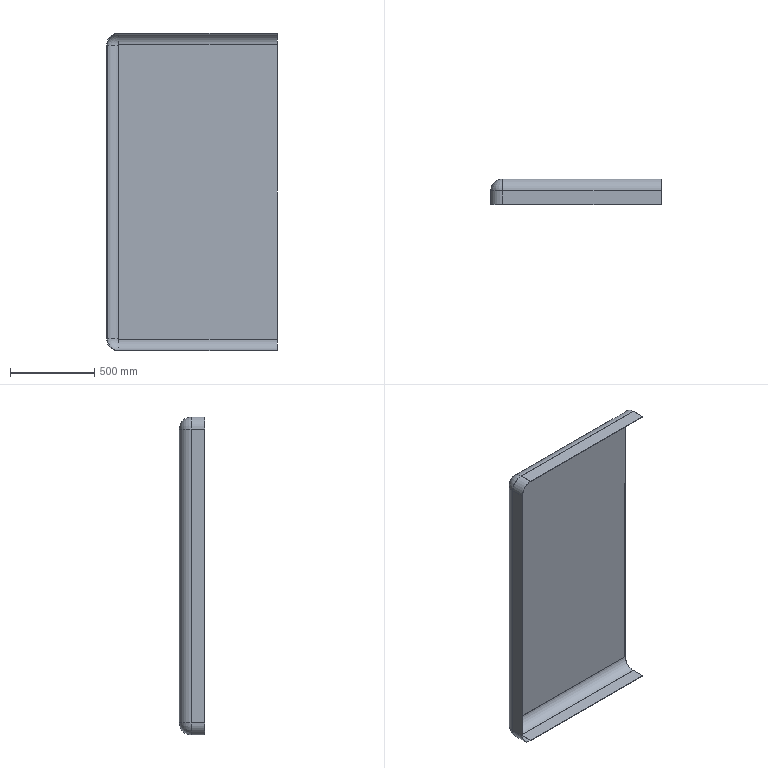Component | SolidWorks | TopHousingAssembly-1_CasingA-1 | 1 solid | 28 faces | box 1009.5 x 149.5 x 1881 mm | volume 7036738 mm3 | plane 14 | cylinder 10 | torus 4 | commonest cylinder face diameters 139 x3 133 x3 141 x2 135 x2
STEP:
#1=CARTESIAN_POINT('',(-0.2362,96.791,71.201));
#2=VERTEX_POINT('',#1);
#3=CARTESIAN_POINT('',(-0.2362,96.909,71.201));
#4=VERTEX_POINT('',#3);
#5=CARTESIAN_POINT('',(-0.2362,96.909,71.201));
#6=DIRECTION('',(0.,1.,0.));
#7=VECTOR('',#6,39.37);
#8=LINE('',#5,#7);
#9=EDGE_CURVE('',#2,#4,#8,.T.);
#10=ORIENTED_EDGE('',*,*,#9,.F.);
#11=CARTESIAN_POINT('',(-0.2362,96.791,2.618));
#12=VERTEX_POINT('',#11);
#13=CARTESIAN_POINT('',(-0.2362,96.791,36.909));
#14=DIRECTION('',(0.,0.,-1.));
#15=VECTOR('',#14,39.37);
#16=LINE('',#13,#15);
#17=EDGE_CURVE('',#2,#12,#16,.T.);
#18=ORIENTED_EDGE('',*,*,#17,.T.);
#19=CARTESIAN_POINT('',(-0.2362,96.909,2.618));
#20=VERTEX_POINT('',#19);
#21=CARTESIAN_POINT('',(-0.2362,96.909,2.618));
#22=DIRECTION('',(0.,1.,0.));
#23=VECTOR('',#22,39.37);
#24=LINE('',#21,#23);
#25=EDGE_CURVE('',#12,#20,#24,.T.);
#26=ORIENTED_EDGE('',*,*,#25,.T.);
#27=CARTESIAN_POINT('',(-0.2362,96.909,71.201));
#28=DIRECTION('',(0.,0.,-1.));
#29=VECTOR('',#28,39.37);
#30=LINE('',#27,#29);
#31=EDGE_CURVE('',#4,#20,#30,.T.);
#32=ORIENTED_EDGE('',*,*,#31,.F.);
#33=EDGE_LOOP('',(#10,#18,#26,#32));
#34=FACE_OUTER_BOUND('',#33,.T.);
#35=CARTESIAN_POINT('',(-0.2362,96.909,71.201));
#36=DIRECTION('',(-1.,0.,0.));
#37=DIRECTION('',(0.,0.,-1.));
#38=AXIS2_PLACEMENT_3D('',#35,#36,#37);
#39=PLANE('',#38);
#40=ADVANCED_FACE('',(#34),#39,.F.);
#41=CARTESIAN_POINT('',(-37.244,96.909,2.657));
#42=VERTEX_POINT('',#41);
#43=CARTESIAN_POINT('',(-37.244,96.909,71.161));
#44=VERTEX_POINT('',#43);
#45=CARTESIAN_POINT('',(-37.244,96.909,71.201));
#46=DIRECTION('',(0.,0.,1.));
#47=VECTOR('',#46,39.37);
#48=LINE('',#45,#47);
#49=EDGE_CURVE('',#42,#44,#48,.T.);
#50=ORIENTED_EDGE('',*,*,#49,.T.);
#51=CARTESIAN_POINT('',(-37.205,96.909,71.201));
#52=VERTEX_POINT('',#51);
#53=CARTESIAN_POINT('',(-37.205,96.909,71.161));
#54=DIRECTION('',(0.,1.,0.));
#55=DIRECTION('',(0.,0.,-1.));
#56=AXIS2_PLACEMENT_3D('',#53,#54,#55);
#57=CIRCLE('',#56,0.03937);
#58=EDGE_CURVE('',#44,#52,#57,.T.);
#59=ORIENTED_EDGE('',*,*,#58,.T.);
#60=CARTESIAN_POINT('',(-37.244,96.909,71.201));
#61=DIRECTION('',(1.,0.,0.));
#62=VECTOR('',#61,39.37);
#63=LINE('',#60,#62);
#64=EDGE_CURVE('',#52,#4,#63,.T.);
#65=ORIENTED_EDGE('',*,*,#64,.T.);
#66=ORIENTED_EDGE('',*,*,#31,.T.);
#67=CARTESIAN_POINT('',(-37.205,96.909,2.618));
#68=VERTEX_POINT('',#67);
#69=CARTESIAN_POINT('',(-37.244,96.909,2.618));
#70=DIRECTION('',(-1.,0.,0.));
#71=VECTOR('',#70,39.37);
#72=LINE('',#69,#71);
#73=EDGE_CURVE('',#20,#68,#72,.T.);
#74=ORIENTED_EDGE('',*,*,#73,.T.);
#75=CARTESIAN_POINT('',(-37.205,96.909,2.657));
#76=DIRECTION('',(0.,1.,0.));
#77=DIRECTION('',(0.,0.,-1.));
#78=AXIS2_PLACEMENT_3D('',#75,#76,#77);
#79=CIRCLE('',#78,0.03937);
#80=EDGE_CURVE('',#68,#42,#79,.T.);
#81=ORIENTED_EDGE('',*,*,#80,.T.);
#82=EDGE_LOOP('',(#50,#59,#65,#66,#74,#81));
#83=FACE_OUTER_BOUND('',#82,.T.);
#84=CARTESIAN_POINT('',(-18.74,96.909,36.909));
#85=DIRECTION('',(0.,-1.,0.));
#86=DIRECTION('',(0.,0.,-1.));
#87=AXIS2_PLACEMENT_3D('',#84,#85,#86);
#88=PLANE('',#87);
#89=ADVANCED_FACE('',(#83),#88,.F.);
#90=CARTESIAN_POINT('',(-37.205,96.791,71.201));
#91=VERTEX_POINT('',#90);
#92=CARTESIAN_POINT('',(-18.74,96.791,71.201));
#93=DIRECTION('',(1.,0.,0.));
#94=VECTOR('',#93,39.37);
#95=LINE('',#92,#94);
#96=EDGE_CURVE('',#91,#2,#95,.T.);
#97=ORIENTED_EDGE('',*,*,#96,.F.);
#98=CARTESIAN_POINT('',(-37.244,96.791,71.161));
#99=VERTEX_POINT('',#98);
#100=CARTESIAN_POINT('',(-37.205,96.791,71.161));
#101=DIRECTION('',(0.,-1.,0.));
#102=DIRECTION('',(0.,0.,-1.));
#103=AXIS2_PLACEMENT_3D('',#100,#101,#102);
#104=CIRCLE('',#103,0.03937);
#105=EDGE_CURVE('',#91,#99,#104,.T.);
#106=ORIENTED_EDGE('',*,*,#105,.T.);
#107=CARTESIAN_POINT('',(-37.244,96.791,2.657));
#108=VERTEX_POINT('',#107);
#109=CARTESIAN_POINT('',(-37.244,96.791,36.909));
#110=DIRECTION('',(0.,0.,1.));
#111=VECTOR('',#110,39.37);
#112=LINE('',#109,#111);
#113=EDGE_CURVE('',#108,#99,#112,.T.);
#114=ORIENTED_EDGE('',*,*,#113,.F.);
#115=CARTESIAN_POINT('',(-37.205,96.791,2.618));
#116=VERTEX_POINT('',#115);
#117=CARTESIAN_POINT('',(-37.205,96.791,2.657));
#118=DIRECTION('',(0.,-1.,0.));
#119=DIRECTION('',(0.,0.,-1.));
#120=AXIS2_PLACEMENT_3D('',#117,#118,#119);
#121=CIRCLE('',#120,0.03937);
#122=EDGE_CURVE('',#108,#116,#121,.T.);
#123=ORIENTED_EDGE('',*,*,#122,.T.);
#124=CARTESIAN_POINT('',(-18.74,96.791,2.618));
#125=DIRECTION('',(-1.,0.,0.));
#126=VECTOR('',#125,39.37);
#127=LINE('',#124,#126);
#128=EDGE_CURVE('',#12,#116,#127,.T.);
#129=ORIENTED_EDGE('',*,*,#128,.F.);
#130=ORIENTED_EDGE('',*,*,#17,.F.);
#131=EDGE_LOOP('',(#97,#106,#114,#123,#129,#130));
#132=FACE_OUTER_BOUND('',#131,.T.);
#133=CARTESIAN_POINT('',(-18.74,96.791,36.909));
#134=DIRECTION('',(0.,-1.,0.));
#135=DIRECTION('',(0.,0.,-1.));
#136=AXIS2_PLACEMENT_3D('',#133,#134,#135);
#137=PLANE('',#136);
#138=ADVANCED_FACE('',(#132),#137,.T.);
#139=CARTESIAN_POINT('',(-0.2362,94.173,73.819));
#140=VERTEX_POINT('',#139);
#141=CARTESIAN_POINT('',(-0.2362,94.173,73.937));
#142=VERTEX_POINT('',#141);
#143=CARTESIAN_POINT('',(-0.2362,94.173,73.937));
#144=DIRECTION('',(0.,0.,1.));
#145=VECTOR('',#144,39.37);
#146=LINE('',#143,#145);
#147=EDGE_CURVE('',#140,#142,#146,.T.);
#148=ORIENTED_EDGE('',*,*,#147,.F.);
#149=CARTESIAN_POINT('',(-0.2362,94.173,71.201));
#150=DIRECTION('',(1.,0.,0.));
#151=DIRECTION('',(0.,-0.,1.));
#152=AXIS2_PLACEMENT_3D('',#149,#150,#151);
#153=CIRCLE('',#152,2.618);
#154=EDGE_CURVE('',#2,#140,#153,.T.);
#155=ORIENTED_EDGE('',*,*,#154,.F.);
#156=ORIENTED_EDGE('',*,*,#9,.T.);
#157=CARTESIAN_POINT('',(-0.2362,94.173,71.201));
#158=DIRECTION('',(1.,0.,0.));
#159=DIRECTION('',(0.,-0.,1.));
#160=AXIS2_PLACEMENT_3D('',#157,#158,#159);
#161=CIRCLE('',#160,2.736);
#162=EDGE_CURVE('',#4,#142,#161,.T.);
#163=ORIENTED_EDGE('',*,*,#162,.T.);
#164=EDGE_LOOP('',(#148,#155,#156,#163));
#165=FACE_OUTER_BOUND('',#164,.T.);
#166=CARTESIAN_POINT('',(-0.2362,94.173,71.201));
#167=DIRECTION('',(1.,0.,0.));
#168=DIRECTION('',(0.,0.,-1.));
#169=AXIS2_PLACEMENT_3D('',#166,#167,#168);
#170=PLANE('',#169);
#171=ADVANCED_FACE('',(#165),#170,.T.);
#172=ORIENTED_EDGE('',*,*,#64,.F.);
#173=CARTESIAN_POINT('',(-37.205,94.173,73.937));
#174=VERTEX_POINT('',#173);
#175=CARTESIAN_POINT('',(-37.205,94.173,71.201));
#176=DIRECTION('',(-1.,0.,0.));
#177=DIRECTION('',(0.,0.,1.));
#178=AXIS2_PLACEMENT_3D('',#175,#176,#177);
#179=CIRCLE('',#178,2.736);
#180=EDGE_CURVE('',#174,#52,#179,.T.);
#181=ORIENTED_EDGE('',*,*,#180,.F.);
#182=CARTESIAN_POINT('',(-0.2362,94.173,73.937));
#183=DIRECTION('',(1.,0.,0.));
#184=VECTOR('',#183,39.37);
#185=LINE('',#182,#184);
#186=EDGE_CURVE('',#174,#142,#185,.T.);
#187=ORIENTED_EDGE('',*,*,#186,.T.);
#188=ORIENTED_EDGE('',*,*,#162,.F.);
#189=EDGE_LOOP('',(#172,#181,#187,#188));
#190=FACE_OUTER_BOUND('',#189,.T.);
#191=CARTESIAN_POINT('',(-37.205,94.173,71.201));
#192=DIRECTION('',(-1.,0.,0.));
#193=DIRECTION('',(0.,0.,1.));
#194=AXIS2_PLACEMENT_3D('',#191,#192,#193);
#195=CYLINDRICAL_SURFACE('',#194,2.736);
#196=ADVANCED_FACE('',(#190),#195,.T.);
#197=ORIENTED_EDGE('',*,*,#96,.T.);
#198=ORIENTED_EDGE('',*,*,#154,.T.);
#199=CARTESIAN_POINT('',(-37.205,94.173,73.819));
#200=VERTEX_POINT('',#199);
#201=CARTESIAN_POINT('',(-0.2362,94.173,73.819));
#202=DIRECTION('',(-1.,0.,0.));
#203=VECTOR('',#202,39.37);
#204=LINE('',#201,#203);
#205=EDGE_CURVE('',#140,#200,#204,.T.);
#206=ORIENTED_EDGE('',*,*,#205,.T.);
#207=CARTESIAN_POINT('',(-37.205,94.173,71.201));
#208=DIRECTION('',(-1.,0.,0.));
#209=DIRECTION('',(0.,0.,1.));
#210=AXIS2_PLACEMENT_3D('',#207,#208,#209);
#211=CIRCLE('',#210,2.618);
#212=EDGE_CURVE('',#200,#91,#211,.T.);
#213=ORIENTED_EDGE('',*,*,#212,.T.);
#214=EDGE_LOOP('',(#197,#198,#206,#213));
#215=FACE_OUTER_BOUND('',#214,.T.);
#216=CARTESIAN_POINT('',(-37.205,94.173,71.201));
#217=DIRECTION('',(-1.,0.,0.));
#218=DIRECTION('',(0.,0.,1.));
#219=AXIS2_PLACEMENT_3D('',#216,#217,#218);
#220=CYLINDRICAL_SURFACE('',#219,2.618);
#221=ADVANCED_FACE('',(#215),#220,.F.);
#222=ORIENTED_EDGE('',*,*,#147,.T.);
#223=CARTESIAN_POINT('',(-0.2362,91.024,73.937));
#224=VERTEX_POINT('',#223);
#225=CARTESIAN_POINT('',(-0.2362,96.791,73.937));
#226=DIRECTION('',(-0.,1.,-0.));
#227=VECTOR('',#226,39.37);
#228=LINE('',#225,#227);
#229=EDGE_CURVE('',#224,#142,#228,.T.);
#230=ORIENTED_EDGE('',*,*,#229,.F.);
#231=CARTESIAN_POINT('',(-0.2362,91.024,73.819));
#232=VERTEX_POINT('',#231);
#233=CARTESIAN_POINT('',(-0.2362,91.024,73.937));
#234=DIRECTION('',(0.,-0.,-1.));
#235=VECTOR('',#234,39.37);
#236=LINE('',#233,#235);
#237=EDGE_CURVE('',#224,#232,#236,.T.);
#238=ORIENTED_EDGE('',*,*,#237,.T.);
#239=CARTESIAN_POINT('',(-0.2362,96.791,73.819));
#240=DIRECTION('',(-0.,1.,-0.));
#241=VECTOR('',#240,39.37);
#242=LINE('',#239,#241);
#243=EDGE_CURVE('',#232,#140,#242,.T.);
#244=ORIENTED_EDGE('',*,*,#243,.T.);
#245=EDGE_LOOP('',(#222,#230,#238,#244));
#246=FACE_OUTER_BOUND('',#245,.T.);
#247=CARTESIAN_POINT('',(-0.2362,96.791,73.937));
#248=DIRECTION('',(-1.,-0.,0.));
#249=DIRECTION('',(0.,-1.,0.));
#250=AXIS2_PLACEMENT_3D('',#247,#248,#249);
#251=PLANE('',#250);
#252=ADVANCED_FACE('',(#246),#251,.F.);
#253=ORIENTED_EDGE('',*,*,#186,.F.);
#254=CARTESIAN_POINT('',(-37.205,91.024,73.937));
#255=VERTEX_POINT('',#254);
#256=CARTESIAN_POINT('',(-37.205,96.791,73.937));
#257=DIRECTION('',(0.,-1.,0.));
#258=VECTOR('',#257,39.37);
#259=LINE('',#256,#258);
#260=EDGE_CURVE('',#174,#255,#259,.T.);
#261=ORIENTED_EDGE('',*,*,#260,.T.);
#262=CARTESIAN_POINT('',(-18.74,91.024,73.937));
#263=DIRECTION('',(1.,0.,0.));
#264=VECTOR('',#263,39.37);
#265=LINE('',#262,#264);
#266=EDGE_CURVE('',#255,#224,#265,.T.);
#267=ORIENTED_EDGE('',*,*,#266,.T.);
#268=ORIENTED_EDGE('',*,*,#229,.T.);
#269=EDGE_LOOP('',(#253,#261,#267,#268));
#270=FACE_OUTER_BOUND('',#269,.T.);
#271=CARTESIAN_POINT('',(-18.74,96.791,73.937));
#272=DIRECTION('',(0.,-0.,-1.));
#273=DIRECTION('',(0.,1.,-0.));
#274=AXIS2_PLACEMENT_3D('',#271,#272,#273);
#275=PLANE('',#274);
#276=ADVANCED_FACE('',(#270),#275,.F.);
#277=CARTESIAN_POINT('',(-37.205,91.024,73.819));
#278=VERTEX_POINT('',#277);
#279=CARTESIAN_POINT('',(-37.205,91.024,73.819));
#280=DIRECTION('',(0.,-1.,0.));
#281=VECTOR('',#280,39.37);
#282=LINE('',#279,#281);
#283=EDGE_CURVE('',#200,#278,#282,.T.);
#284=ORIENTED_EDGE('',*,*,#283,.F.);
#285=ORIENTED_EDGE('',*,*,#205,.F.);
#286=ORIENTED_EDGE('',*,*,#243,.F.);
#287=CARTESIAN_POINT('',(-0.2362,91.024,73.819));
#288=DIRECTION('',(1.,0.,0.));
#289=VECTOR('',#288,39.37);
#290=LINE('',#287,#289);
#291=EDGE_CURVE('',#278,#232,#290,.T.);
#292=ORIENTED_EDGE('',*,*,#291,.F.);
#293=EDGE_LOOP('',(#284,#285,#286,#292));
#294=FACE_OUTER_BOUND('',#293,.T.);
#295=CARTESIAN_POINT('',(-18.74,96.791,73.819));
#296=DIRECTION('',(0.,-0.,-1.));
#297=DIRECTION('',(0.,1.,-0.));
#298=AXIS2_PLACEMENT_3D('',#295,#296,#297);
#299=PLANE('',#298);
#300=ADVANCED_FACE('',(#294),#299,.T.);
#301=ORIENTED_EDGE('',*,*,#291,.T.);
#302=ORIENTED_EDGE('',*,*,#237,.F.);
#303=ORIENTED_EDGE('',*,*,#266,.F.);
#304=CARTESIAN_POINT('',(-39.98,91.024,71.161));
#305=VERTEX_POINT('',#304);
#306=CARTESIAN_POINT('',(-37.205,91.024,71.161));
#307=DIRECTION('',(0.,-1.,0.));
#308=DIRECTION('',(0.,0.,1.));
#309=AXIS2_PLACEMENT_3D('',#306,#307,#308);
#310=CIRCLE('',#309,2.776);
#311=EDGE_CURVE('',#255,#305,#310,.T.);
#312=ORIENTED_EDGE('',*,*,#311,.T.);
#313=CARTESIAN_POINT('',(-39.98,91.024,2.657));
#314=VERTEX_POINT('',#313);
#315=CARTESIAN_POINT('',(-39.98,91.024,36.909));
#316=DIRECTION('',(0.,0.,1.));
#317=VECTOR('',#316,39.37);
#318=LINE('',#315,#317);
#319=EDGE_CURVE('',#314,#305,#318,.T.);
#320=ORIENTED_EDGE('',*,*,#319,.F.);
#321=CARTESIAN_POINT('',(-37.205,91.024,-0.1181));
#322=VERTEX_POINT('',#321);
#323=CARTESIAN_POINT('',(-37.205,91.024,2.657));
#324=DIRECTION('',(0.,-1.,0.));
#325=DIRECTION('',(-1.,0.,0.));
#326=AXIS2_PLACEMENT_3D('',#323,#324,#325);
#327=CIRCLE('',#326,2.776);
#328=EDGE_CURVE('',#314,#322,#327,.T.);
#329=ORIENTED_EDGE('',*,*,#328,.T.);
#330=CARTESIAN_POINT('',(-0.2362,91.024,-0.1181));
#331=VERTEX_POINT('',#330);
#332=CARTESIAN_POINT('',(-18.74,91.024,-0.1181));
#333=DIRECTION('',(-1.,0.,0.));
#334=VECTOR('',#333,39.37);
#335=LINE('',#332,#334);
#336=EDGE_CURVE('',#331,#322,#335,.T.);
#337=ORIENTED_EDGE('',*,*,#336,.F.);
#338=CARTESIAN_POINT('',(-0.2362,91.024,-0.));
#339=VERTEX_POINT('',#338);
#340=CARTESIAN_POINT('',(-0.2362,91.024,-0.1181));
#341=DIRECTION('',(0.,-0.,1.));
#342=VECTOR('',#341,39.37);
#343=LINE('',#340,#342);
#344=EDGE_CURVE('',#331,#339,#343,.T.);
#345=ORIENTED_EDGE('',*,*,#344,.T.);
#346=CARTESIAN_POINT('',(-37.205,91.024,-0.));
#347=VERTEX_POINT('',#346);
#348=CARTESIAN_POINT('',(-37.205,91.024,-0.));
#349=DIRECTION('',(-1.,0.,0.));
#350=VECTOR('',#349,39.37);
#351=LINE('',#348,#350);
#352=EDGE_CURVE('',#339,#347,#351,.T.);
#353=ORIENTED_EDGE('',*,*,#352,.T.);
#354=CARTESIAN_POINT('',(-39.862,91.024,2.657));
#355=VERTEX_POINT('',#354);
#356=CARTESIAN_POINT('',(-37.205,91.024,2.657));
#357=DIRECTION('',(0.,-1.,0.));
#358=DIRECTION('',(-1.,0.,0.));
#359=AXIS2_PLACEMENT_3D('',#356,#357,#358);
#360=CIRCLE('',#359,2.657);
#361=EDGE_CURVE('',#355,#347,#360,.T.);
#362=ORIENTED_EDGE('',*,*,#361,.F.);
#363=CARTESIAN_POINT('',(-39.862,91.024,71.161));
#364=VERTEX_POINT('',#363);
#365=CARTESIAN_POINT('',(-39.862,91.024,71.161));
#366=DIRECTION('',(0.,0.,1.));
#367=VECTOR('',#366,39.37);
#368=LINE('',#365,#367);
#369=EDGE_CURVE('',#355,#364,#368,.T.);
#370=ORIENTED_EDGE('',*,*,#369,.T.);
#371=CARTESIAN_POINT('',(-37.205,91.024,71.161));
#372=DIRECTION('',(0.,-1.,0.));
#373=DIRECTION('',(0.,0.,1.));
#374=AXIS2_PLACEMENT_3D('',#371,#372,#373);
#375=CIRCLE('',#374,2.657);
#376=EDGE_CURVE('',#278,#364,#375,.T.);
#377=ORIENTED_EDGE('',*,*,#376,.F.);
#378=EDGE_LOOP('',(#301,#302,#303,#312,#320,#329,#337,#345,#353,#362,#370,#377));
#379=FACE_OUTER_BOUND('',#378,.T.);
#380=CARTESIAN_POINT('',(-0.2362,91.024,73.937));
#381=DIRECTION('',(0.,1.,-0.));
#382=DIRECTION('',(0.,0.,1.));
#383=AXIS2_PLACEMENT_3D('',#380,#381,#382);
#384=PLANE('',#383);
#385=ADVANCED_FACE('',(#379),#384,.F.);
#386=ORIENTED_EDGE('',*,*,#49,.F.);
#387=CARTESIAN_POINT('',(-39.98,94.173,2.657));
#388=VERTEX_POINT('',#387);
#389=CARTESIAN_POINT('',(-37.244,94.173,2.657));
#390=DIRECTION('',(0.,0.,-1.));
#391=DIRECTION('',(-1.,0.,0.));
#392=AXIS2_PLACEMENT_3D('',#389,#390,#391);
#393=CIRCLE('',#392,2.736);
#394=EDGE_CURVE('',#388,#42,#393,.T.);
#395=ORIENTED_EDGE('',*,*,#394,.F.);
#396=CARTESIAN_POINT('',(-39.98,94.173,71.161));
#397=VERTEX_POINT('',#396);
#398=CARTESIAN_POINT('',(-39.98,94.173,71.161));
#399=DIRECTION('',(0.,0.,1.));
#400=VECTOR('',#399,39.37);
#401=LINE('',#398,#400);
#402=EDGE_CURVE('',#388,#397,#401,.T.);
#403=ORIENTED_EDGE('',*,*,#402,.T.);
#404=CARTESIAN_POINT('',(-37.244,94.173,71.161));
#405=DIRECTION('',(0.,0.,1.));
#406=DIRECTION('',(-1.,-0.,0.));
#407=AXIS2_PLACEMENT_3D('',#404,#405,#406);
#408=CIRCLE('',#407,2.736);
#409=EDGE_CURVE('',#44,#397,#408,.T.);
#410=ORIENTED_EDGE('',*,*,#409,.F.);
#411=EDGE_LOOP('',(#386,#395,#403,#410));
#412=FACE_OUTER_BOUND('',#411,.T.);
#413=CARTESIAN_POINT('',(-37.244,94.173,2.657));
#414=DIRECTION('',(0.,0.,-1.));
#415=DIRECTION('',(-1.,0.,0.));
#416=AXIS2_PLACEMENT_3D('',#413,#414,#415);
#417=CYLINDRICAL_SURFACE('',#416,2.736);
#418=ADVANCED_FACE('',(#412),#417,.T.);
#419=ORIENTED_EDGE('',*,*,#113,.T.);
#420=CARTESIAN_POINT('',(-39.862,94.173,71.161));
#421=VERTEX_POINT('',#420);
#422=CARTESIAN_POINT('',(-37.244,94.173,71.161));
#423=DIRECTION('',(0.,0.,1.));
#424=DIRECTION('',(-1.,0.,0.));
#425=AXIS2_PLACEMENT_3D('',#422,#423,#424);
#426=CIRCLE('',#425,2.618);
#427=EDGE_CURVE('',#99,#421,#426,.T.);
#428=ORIENTED_EDGE('',*,*,#427,.T.);
#429=CARTESIAN_POINT('',(-39.862,94.173,2.657));
#430=VERTEX_POINT('',#429);
#431=CARTESIAN_POINT('',(-39.862,94.173,71.161));
#432=DIRECTION('',(0.,0.,-1.));
#433=VECTOR('',#432,39.37);
#434=LINE('',#431,#433);
#435=EDGE_CURVE('',#421,#430,#434,.T.);
#436=ORIENTED_EDGE('',*,*,#435,.T.);
#437=CARTESIAN_POINT('',(-37.244,94.173,2.657));
#438=DIRECTION('',(0.,0.,-1.));
#439=DIRECTION('',(-1.,0.,0.));
#440=AXIS2_PLACEMENT_3D('',#437,#438,#439);
#441=CIRCLE('',#440,2.618);
#442=EDGE_CURVE('',#430,#108,#441,.T.);
#443=ORIENTED_EDGE('',*,*,#442,.T.);
#444=EDGE_LOOP('',(#419,#428,#436,#443));
#445=FACE_OUTER_BOUND('',#444,.T.);
#446=CARTESIAN_POINT('',(-37.244,94.173,2.657));
#447=DIRECTION('',(0.,0.,-1.));
#448=DIRECTION('',(-1.,0.,0.));
#449=AXIS2_PLACEMENT_3D('',#446,#447,#448);
#450=CYLINDRICAL_SURFACE('',#449,2.618);
#451=ADVANCED_FACE('',(#445),#450,.F.);
#452=ORIENTED_EDGE('',*,*,#402,.F.);
#453=CARTESIAN_POINT('',(-39.98,96.791,2.657));
#454=DIRECTION('',(-0.,-1.,0.));
#455=VECTOR('',#454,39.37);
#456=LINE('',#453,#455);
#457=EDGE_CURVE('',#388,#314,#456,.T.);
#458=ORIENTED_EDGE('',*,*,#457,.T.);
#459=ORIENTED_EDGE('',*,*,#319,.T.);
#460=CARTESIAN_POINT('',(-39.98,96.791,71.161));
#461=DIRECTION('',(0.,1.,0.));
#462=VECTOR('',#461,39.37);
#463=LINE('',#460,#462);
#464=EDGE_CURVE('',#305,#397,#463,.T.);
#465=ORIENTED_EDGE('',*,*,#464,.T.);
#466=EDGE_LOOP('',(#452,#458,#459,#465));
#467=FACE_OUTER_BOUND('',#466,.T.);
#468=CARTESIAN_POINT('',(-39.98,96.791,36.909));
#469=DIRECTION('',(1.,-0.,0.));
#470=DIRECTION('',(0.,1.,0.));
#471=AXIS2_PLACEMENT_3D('',#468,#469,#470);
#472=PLANE('',#471);
#473=ADVANCED_FACE('',(#467),#472,.F.);
#474=CARTESIAN_POINT('',(-39.862,91.024,2.657));
#475=DIRECTION('',(-0.,-1.,0.));
#476=VECTOR('',#475,39.37);
#477=LINE('',#474,#476);
#478=EDGE_CURVE('',#430,#355,#477,.T.);
#479=ORIENTED_EDGE('',*,*,#478,.F.);
#480=ORIENTED_EDGE('',*,*,#435,.F.);
#481=CARTESIAN_POINT('',(-39.862,96.791,71.161));
#482=DIRECTION('',(0.,1.,0.));
#483=VECTOR('',#482,39.37);
#484=LINE('',#481,#483);
#485=EDGE_CURVE('',#364,#421,#484,.T.);
#486=ORIENTED_EDGE('',*,*,#485,.F.);
#487=ORIENTED_EDGE('',*,*,#369,.F.);
#488=EDGE_LOOP('',(#479,#480,#486,#487));
#489=FACE_OUTER_BOUND('',#488,.T.);
#490=CARTESIAN_POINT('',(-39.862,96.791,36.909));
#491=DIRECTION('',(1.,-0.,0.));
#492=DIRECTION('',(0.,1.,0.));
#493=AXIS2_PLACEMENT_3D('',#490,#491,#492);
#494=PLANE('',#493);
#495=ADVANCED_FACE('',(#489),#494,.T.);
#496=CARTESIAN_POINT('',(-0.2362,94.173,-0.));
#497=VERTEX_POINT('',#496);
#498=CARTESIAN_POINT('',(-0.2362,94.173,2.618));
#499=DIRECTION('',(1.,0.,0.));
#500=DIRECTION('',(0.,0.,-1.));
#501=AXIS2_PLACEMENT_3D('',#498,#499,#500);
#502=CIRCLE('',#501,2.618);
#503=EDGE_CURVE('',#497,#12,#502,.T.);
#504=ORIENTED_EDGE('',*,*,#503,.F.);
#505=CARTESIAN_POINT('',(-0.2362,94.173,-0.1181));
#506=VERTEX_POINT('',#505);
#507=CARTESIAN_POINT('',(-0.2362,94.173,-0.));
#508=DIRECTION('',(0.,0.,-1.));
#509=VECTOR('',#508,39.37);
#510=LINE('',#507,#509);
#511=EDGE_CURVE('',#497,#506,#510,.T.);
#512=ORIENTED_EDGE('',*,*,#511,.T.);
#513=CARTESIAN_POINT('',(-0.2362,94.173,2.618));
#514=DIRECTION('',(1.,0.,0.));
#515=DIRECTION('',(0.,0.,-1.));
#516=AXIS2_PLACEMENT_3D('',#513,#514,#515);
#517=CIRCLE('',#516,2.736);
#518=EDGE_CURVE('',#506,#20,#517,.T.);
#519=ORIENTED_EDGE('',*,*,#518,.T.);
#520=ORIENTED_EDGE('',*,*,#25,.F.);
#521=EDGE_LOOP('',(#504,#512,#519,#520));
#522=FACE_OUTER_BOUND('',#521,.T.);
#523=CARTESIAN_POINT('',(-0.2362,94.173,2.618));
#524=DIRECTION('',(-1.,0.,0.));
#525=DIRECTION('',(0.,0.,1.));
#526=AXIS2_PLACEMENT_3D('',#523,#524,#525);
#527=PLANE('',#526);
#528=ADVANCED_FACE('',(#522),#527,.F.);
#529=ORIENTED_EDGE('',*,*,#73,.F.);
#530=ORIENTED_EDGE('',*,*,#518,.F.);
#531=CARTESIAN_POINT('',(-37.205,94.173,-0.1181));
#532=VERTEX_POINT('',#531);
#533=CARTESIAN_POINT('',(-37.205,94.173,-0.1181));
#534=DIRECTION('',(-1.,0.,0.));
#535=VECTOR('',#534,39.37);
#536=LINE('',#533,#535);
#537=EDGE_CURVE('',#506,#532,#536,.T.);
#538=ORIENTED_EDGE('',*,*,#537,.T.);
#539=CARTESIAN_POINT('',(-37.205,94.173,2.618));
#540=DIRECTION('',(-1.,0.,0.));
#541=DIRECTION('',(0.,-0.,-1.));
#542=AXIS2_PLACEMENT_3D('',#539,#540,#541);
#543=CIRCLE('',#542,2.736);
#544=EDGE_CURVE('',#68,#532,#543,.T.);
#545=ORIENTED_EDGE('',*,*,#544,.F.);
#546=EDGE_LOOP('',(#529,#530,#538,#545));
#547=FACE_OUTER_BOUND('',#546,.T.);
#548=CARTESIAN_POINT('',(-0.2362,94.173,2.618));
#549=DIRECTION('',(1.,0.,0.));
#550=DIRECTION('',(0.,0.,-1.));
#551=AXIS2_PLACEMENT_3D('',#548,#549,#550);
#552=CYLINDRICAL_SURFACE('',#551,2.736);
#553=ADVANCED_FACE('',(#547),#552,.T.);
#554=ORIENTED_EDGE('',*,*,#128,.T.);
#555=CARTESIAN_POINT('',(-37.205,94.173,-0.));
#556=VERTEX_POINT('',#555);
#557=CARTESIAN_POINT('',(-37.205,94.173,2.618));
#558=DIRECTION('',(-1.,0.,0.));
#559=DIRECTION('',(0.,-0.,-1.));
#560=AXIS2_PLACEMENT_3D('',#557,#558,#559);
#561=CIRCLE('',#560,2.618);
#562=EDGE_CURVE('',#116,#556,#561,.T.);
#563=ORIENTED_EDGE('',*,*,#562,.T.);
#564=CARTESIAN_POINT('',(-37.205,94.173,-0.));
#565=DIRECTION('',(1.,0.,0.));
#566=VECTOR('',#565,39.37);
#567=LINE('',#564,#566);
#568=EDGE_CURVE('',#556,#497,#567,.T.);
#569=ORIENTED_EDGE('',*,*,#568,.T.);
#570=ORIENTED_EDGE('',*,*,#503,.T.);
#571=EDGE_LOOP('',(#554,#563,#569,#570));
#572=FACE_OUTER_BOUND('',#571,.T.);
#573=CARTESIAN_POINT('',(-0.2362,94.173,2.618));
#574=DIRECTION('',(1.,0.,0.));
#575=DIRECTION('',(0.,0.,-1.));
#576=AXIS2_PLACEMENT_3D('',#573,#574,#575);
#577=CYLINDRICAL_SURFACE('',#576,2.618);
#578=ADVANCED_FACE('',(#572),#577,.F.);
#579=ORIENTED_EDGE('',*,*,#511,.F.);
#580=CARTESIAN_POINT('',(-0.2362,91.024,-0.));
#581=DIRECTION('',(-0.,-1.,-0.));
#582=VECTOR('',#581,39.37);
#583=LINE('',#580,#582);
#584=EDGE_CURVE('',#497,#339,#583,.T.);
#585=ORIENTED_EDGE('',*,*,#584,.T.);
#586=ORIENTED_EDGE('',*,*,#344,.F.);
#587=CARTESIAN_POINT('',(-0.2362,96.791,-0.1181));
#588=DIRECTION('',(-0.,-1.,-0.));
#589=VECTOR('',#588,39.37);
#590=LINE('',#587,#589);
#591=EDGE_CURVE('',#506,#331,#590,.T.);
#592=ORIENTED_EDGE('',*,*,#591,.F.);
#593=EDGE_LOOP('',(#579,#585,#586,#592));
#594=FACE_OUTER_BOUND('',#593,.T.);
#595=CARTESIAN_POINT('',(-0.2362,91.024,-0.1181));
#596=DIRECTION('',(-1.,0.,0.));
#597=DIRECTION('',(-0.,-1.,0.));
#598=AXIS2_PLACEMENT_3D('',#595,#596,#597);
#599=PLANE('',#598);
#600=ADVANCED_FACE('',(#594),#599,.F.);
#601=ORIENTED_EDGE('',*,*,#537,.F.);
#602=ORIENTED_EDGE('',*,*,#591,.T.);
#603=ORIENTED_EDGE('',*,*,#336,.T.);
#604=CARTESIAN_POINT('',(-37.205,96.791,-0.1181));
#605=DIRECTION('',(0.,1.,0.));
#606=VECTOR('',#605,39.37);
#607=LINE('',#604,#606);
#608=EDGE_CURVE('',#322,#532,#607,.T.);
#609=ORIENTED_EDGE('',*,*,#608,.T.);
#610=EDGE_LOOP('',(#601,#602,#603,#609));
#611=FACE_OUTER_BOUND('',#610,.T.);
#612=CARTESIAN_POINT('',(-18.74,96.791,-0.1181));
#613=DIRECTION('',(0.,-0.,1.));
#614=DIRECTION('',(0.,-1.,-0.));
#615=AXIS2_PLACEMENT_3D('',#612,#613,#614);
#616=PLANE('',#615);
#617=ADVANCED_FACE('',(#611),#616,.F.);
#618=ORIENTED_EDGE('',*,*,#584,.F.);
#619=ORIENTED_EDGE('',*,*,#568,.F.);
#620=CARTESIAN_POINT('',(-37.205,96.791,-0.));
#621=DIRECTION('',(0.,1.,0.));
#622=VECTOR('',#621,39.37);
#623=LINE('',#620,#622);
#624=EDGE_CURVE('',#347,#556,#623,.T.);
#625=ORIENTED_EDGE('',*,*,#624,.F.);
#626=ORIENTED_EDGE('',*,*,#352,.F.);
#627=EDGE_LOOP('',(#618,#619,#625,#626));
#628=FACE_OUTER_BOUND('',#627,.T.);
#629=CARTESIAN_POINT('',(-18.74,96.791,-0.));
#630=DIRECTION('',(0.,-0.,1.));
#631=DIRECTION('',(0.,-1.,-0.));
#632=AXIS2_PLACEMENT_3D('',#629,#630,#631);
#633=PLANE('',#632);
#634=ADVANCED_FACE('',(#628),#633,.T.);
#635=ORIENTED_EDGE('',*,*,#105,.F.);
#636=ORIENTED_EDGE('',*,*,#212,.F.);
#637=CARTESIAN_POINT('',(-37.205,94.173,71.161));
#638=DIRECTION('',(0.,-1.,0.));
#639=DIRECTION('',(0.,0.,1.));
#640=AXIS2_PLACEMENT_3D('',#637,#638,#639);
#641=CIRCLE('',#640,2.657);
#642=EDGE_CURVE('',#200,#421,#641,.T.);
#643=ORIENTED_EDGE('',*,*,#642,.T.);
#644=ORIENTED_EDGE('',*,*,#427,.F.);
#645=EDGE_LOOP('',(#635,#636,#643,#644));
#646=FACE_OUTER_BOUND('',#645,.T.);
#647=CARTESIAN_POINT('',(-37.205,94.173,71.161));
#648=DIRECTION('',(0.,-1.,0.));
#649=DIRECTION('',(0.,0.,-1.));
#650=AXIS2_PLACEMENT_3D('',#647,#648,#649);
#651=TOROIDAL_SURFACE('',#650,0.03937,2.618);
#652=ADVANCED_FACE('',(#646),#651,.F.);
#653=CARTESIAN_POINT('',(-37.205,94.173,71.161));
#654=DIRECTION('',(0.,-1.,0.));
#655=DIRECTION('',(0.,0.,1.));
#656=AXIS2_PLACEMENT_3D('',#653,#654,#655);
#657=CIRCLE('',#656,2.776);
#658=EDGE_CURVE('',#174,#397,#657,.T.);
#659=ORIENTED_EDGE('',*,*,#658,.F.);
#660=ORIENTED_EDGE('',*,*,#180,.T.);
#661=ORIENTED_EDGE('',*,*,#58,.F.);
#662=ORIENTED_EDGE('',*,*,#409,.T.);
#663=EDGE_LOOP('',(#659,#660,#661,#662));
#664=FACE_OUTER_BOUND('',#663,.T.);
#665=CARTESIAN_POINT('',(-37.205,94.173,71.161));
#666=DIRECTION('',(0.,-1.,0.));
#667=DIRECTION('',(0.,0.,-1.));
#668=AXIS2_PLACEMENT_3D('',#665,#666,#667);
#669=TOROIDAL_SURFACE('',#668,0.03937,2.736);
#670=ADVANCED_FACE('',(#664),#669,.T.);
#671=ORIENTED_EDGE('',*,*,#311,.F.);
#672=ORIENTED_EDGE('',*,*,#260,.F.);
#673=ORIENTED_EDGE('',*,*,#658,.T.);
#674=ORIENTED_EDGE('',*,*,#464,.F.);
#675=EDGE_LOOP('',(#671,#672,#673,#674));
#676=FACE_OUTER_BOUND('',#675,.T.);
#677=CARTESIAN_POINT('',(-37.205,94.173,71.161));
#678=DIRECTION('',(0.,-1.,0.));
#679=DIRECTION('',(0.,0.,-1.));
#680=AXIS2_PLACEMENT_3D('',#677,#678,#679);
#681=CYLINDRICAL_SURFACE('',#680,2.776);
#682=ADVANCED_FACE('',(#676),#681,.T.);
#683=ORIENTED_EDGE('',*,*,#642,.F.);
#684=ORIENTED_EDGE('',*,*,#283,.T.);
#685=ORIENTED_EDGE('',*,*,#376,.T.);
#686=ORIENTED_EDGE('',*,*,#485,.T.);
#687=EDGE_LOOP('',(#683,#684,#685,#686));
#688=FACE_OUTER_BOUND('',#687,.T.);
#689=CARTESIAN_POINT('',(-37.205,94.173,71.161));
#690=DIRECTION('',(0.,-1.,0.));
#691=DIRECTION('',(0.,0.,-1.));
#692=AXIS2_PLACEMENT_3D('',#689,#690,#691);
#693=CYLINDRICAL_SURFACE('',#692,2.657);
#694=ADVANCED_FACE('',(#688),#693,.F.);
#695=ORIENTED_EDGE('',*,*,#122,.F.);
#696=ORIENTED_EDGE('',*,*,#442,.F.);
#697=CARTESIAN_POINT('',(-37.205,94.173,2.657));
#698=DIRECTION('',(0.,-1.,0.));
#699=DIRECTION('',(-1.,0.,0.));
#700=AXIS2_PLACEMENT_3D('',#697,#698,#699);
#701=CIRCLE('',#700,2.657);
#702=EDGE_CURVE('',#430,#556,#701,.T.);
#703=ORIENTED_EDGE('',*,*,#702,.T.);
#704=ORIENTED_EDGE('',*,*,#562,.F.);
#705=EDGE_LOOP('',(#695,#696,#703,#704));
#706=FACE_OUTER_BOUND('',#705,.T.);
#707=CARTESIAN_POINT('',(-37.205,94.173,2.657));
#708=DIRECTION('',(0.,-1.,0.));
#709=DIRECTION('',(0.,0.,-1.));
#710=AXIS2_PLACEMENT_3D('',#707,#708,#709);
#711=TOROIDAL_SURFACE('',#710,0.03937,2.618);
#712=ADVANCED_FACE('',(#706),#711,.F.);
#713=CARTESIAN_POINT('',(-37.205,94.173,2.657));
#714=DIRECTION('',(0.,-1.,0.));
#715=DIRECTION('',(-1.,0.,0.));
#716=AXIS2_PLACEMENT_3D('',#713,#714,#715);
#717=CIRCLE('',#716,2.776);
#718=EDGE_CURVE('',#388,#532,#717,.T.);
#719=ORIENTED_EDGE('',*,*,#718,.F.);
#720=ORIENTED_EDGE('',*,*,#394,.T.);
#721=ORIENTED_EDGE('',*,*,#80,.F.);
#722=ORIENTED_EDGE('',*,*,#544,.T.);
#723=EDGE_LOOP('',(#719,#720,#721,#722));
#724=FACE_OUTER_BOUND('',#723,.T.);
#725=CARTESIAN_POINT('',(-37.205,94.173,2.657));
#726=DIRECTION('',(0.,-1.,0.));
#727=DIRECTION('',(0.,0.,-1.));
#728=AXIS2_PLACEMENT_3D('',#725,#726,#727);
#729=TOROIDAL_SURFACE('',#728,0.03937,2.736);
#730=ADVANCED_FACE('',(#724),#729,.T.);
#731=ORIENTED_EDGE('',*,*,#328,.F.);
#732=ORIENTED_EDGE('',*,*,#457,.F.);
#733=ORIENTED_EDGE('',*,*,#718,.T.);
#734=ORIENTED_EDGE('',*,*,#608,.F.);
#735=EDGE_LOOP('',(#731,#732,#733,#734));
#736=FACE_OUTER_BOUND('',#735,.T.);
#737=CARTESIAN_POINT('',(-37.205,94.173,2.657));
#738=DIRECTION('',(0.,-1.,0.));
#739=DIRECTION('',(0.,0.,-1.));
#740=AXIS2_PLACEMENT_3D('',#737,#738,#739);
#741=CYLINDRICAL_SURFACE('',#740,2.776);
#742=ADVANCED_FACE('',(#736),#741,.T.);
#743=ORIENTED_EDGE('',*,*,#702,.F.);
#744=ORIENTED_EDGE('',*,*,#478,.T.);
#745=ORIENTED_EDGE('',*,*,#361,.T.);
#746=ORIENTED_EDGE('',*,*,#624,.T.);
#747=EDGE_LOOP('',(#743,#744,#745,#746));
#748=FACE_OUTER_BOUND('',#747,.T.);
#749=CARTESIAN_POINT('',(-37.205,94.173,2.657));
#750=DIRECTION('',(0.,-1.,0.));
#751=DIRECTION('',(0.,0.,-1.));
#752=AXIS2_PLACEMENT_3D('',#749,#750,#751);
#753=CYLINDRICAL_SURFACE('',#752,2.657);
#754=ADVANCED_FACE('',(#748),#753,.F.);
#755=CLOSED_SHELL('',(#40,#89,#138,#171,#196,#221,#252,#276,#300,#385,#418,#451,#473,#495,#528,#553,#578,#600,#617,#634,#652,#670,#682,#694,#712,#730,#742,#754));
#756=MANIFOLD_SOLID_BREP('',#755);
#757=CARTESIAN_POINT('',(0.,0.,0.));
#758=DIRECTION('',(0.,0.,1.));
#759=DIRECTION('',(1.,0.,0.));
#760=AXIS2_PLACEMENT_3D('',#757,#758,#759);
#761=(LENGTH_UNIT()NAMED_UNIT(*)SI_UNIT($,.METRE.));
#762=LENGTH_MEASURE_WITH_UNIT(LENGTH_MEASURE(0.0254),#761);
#763=DIMENSIONAL_EXPONENTS(1.,0.,0.,0.,0.,0.,0.);
#764=(CONVERSION_BASED_UNIT('',#762)LENGTH_UNIT()NAMED_UNIT(#763));
#765=UNCERTAINTY_MEASURE_WITH_UNIT(LENGTH_MEASURE(0.00001),#764,'','');
#766=(NAMED_UNIT(*)PLANE_ANGLE_UNIT()SI_UNIT($,.RADIAN.));
#767=(NAMED_UNIT(*)SI_UNIT($,.STERADIAN.)SOLID_ANGLE_UNIT());
#768=(GEOMETRIC_REPRESENTATION_CONTEXT(3)GLOBAL_UNCERTAINTY_ASSIGNED_CONTEXT((#765))GLOBAL_UNIT_ASSIGNED_CONTEXT((#764,#766,#767))REPRESENTATION_CONTEXT('',''));
#769=ADVANCED_BREP_SHAPE_REPRESENTATION('',(#756,#760),#768);
#770=COLOUR_RGB('',0.7922,0.8196,0.9333);
#771=FILL_AREA_STYLE_COLOUR('',#770);
#772=FILL_AREA_STYLE('',(#771));
#773=SURFACE_STYLE_FILL_AREA(#772);
#774=SURFACE_SIDE_STYLE('',(#773));
#775=SURFACE_STYLE_USAGE(.BOTH.,#774);
#776=PRESENTATION_STYLE_ASSIGNMENT((#775));
#777=STYLED_ITEM('',(#776),#756);
#778=(LENGTH_UNIT()NAMED_UNIT(*)SI_UNIT($,.METRE.));
#779=LENGTH_MEASURE_WITH_UNIT(LENGTH_MEASURE(0.0254),#778);
#780=DIMENSIONAL_EXPONENTS(1.,0.,0.,0.,0.,0.,0.);
#781=(CONVERSION_BASED_UNIT('',#779)LENGTH_UNIT()NAMED_UNIT(#780));
#782=UNCERTAINTY_MEASURE_WITH_UNIT(LENGTH_MEASURE(0.00001),#781,'','');
#783=(NAMED_UNIT(*)PLANE_ANGLE_UNIT()SI_UNIT($,.RADIAN.));
#784=(NAMED_UNIT(*)SI_UNIT($,.STERADIAN.)SOLID_ANGLE_UNIT());
#785=(GEOMETRIC_REPRESENTATION_CONTEXT(3)GLOBAL_UNCERTAINTY_ASSIGNED_CONTEXT((#782))GLOBAL_UNIT_ASSIGNED_CONTEXT((#781,#783,#784))REPRESENTATION_CONTEXT('',''));
#786=MECHANICAL_DESIGN_GEOMETRIC_PRESENTATION_REPRESENTATION('',(#777),#785);
#787=PRESENTATION_LAYER_ASSIGNMENT('','',(#777));